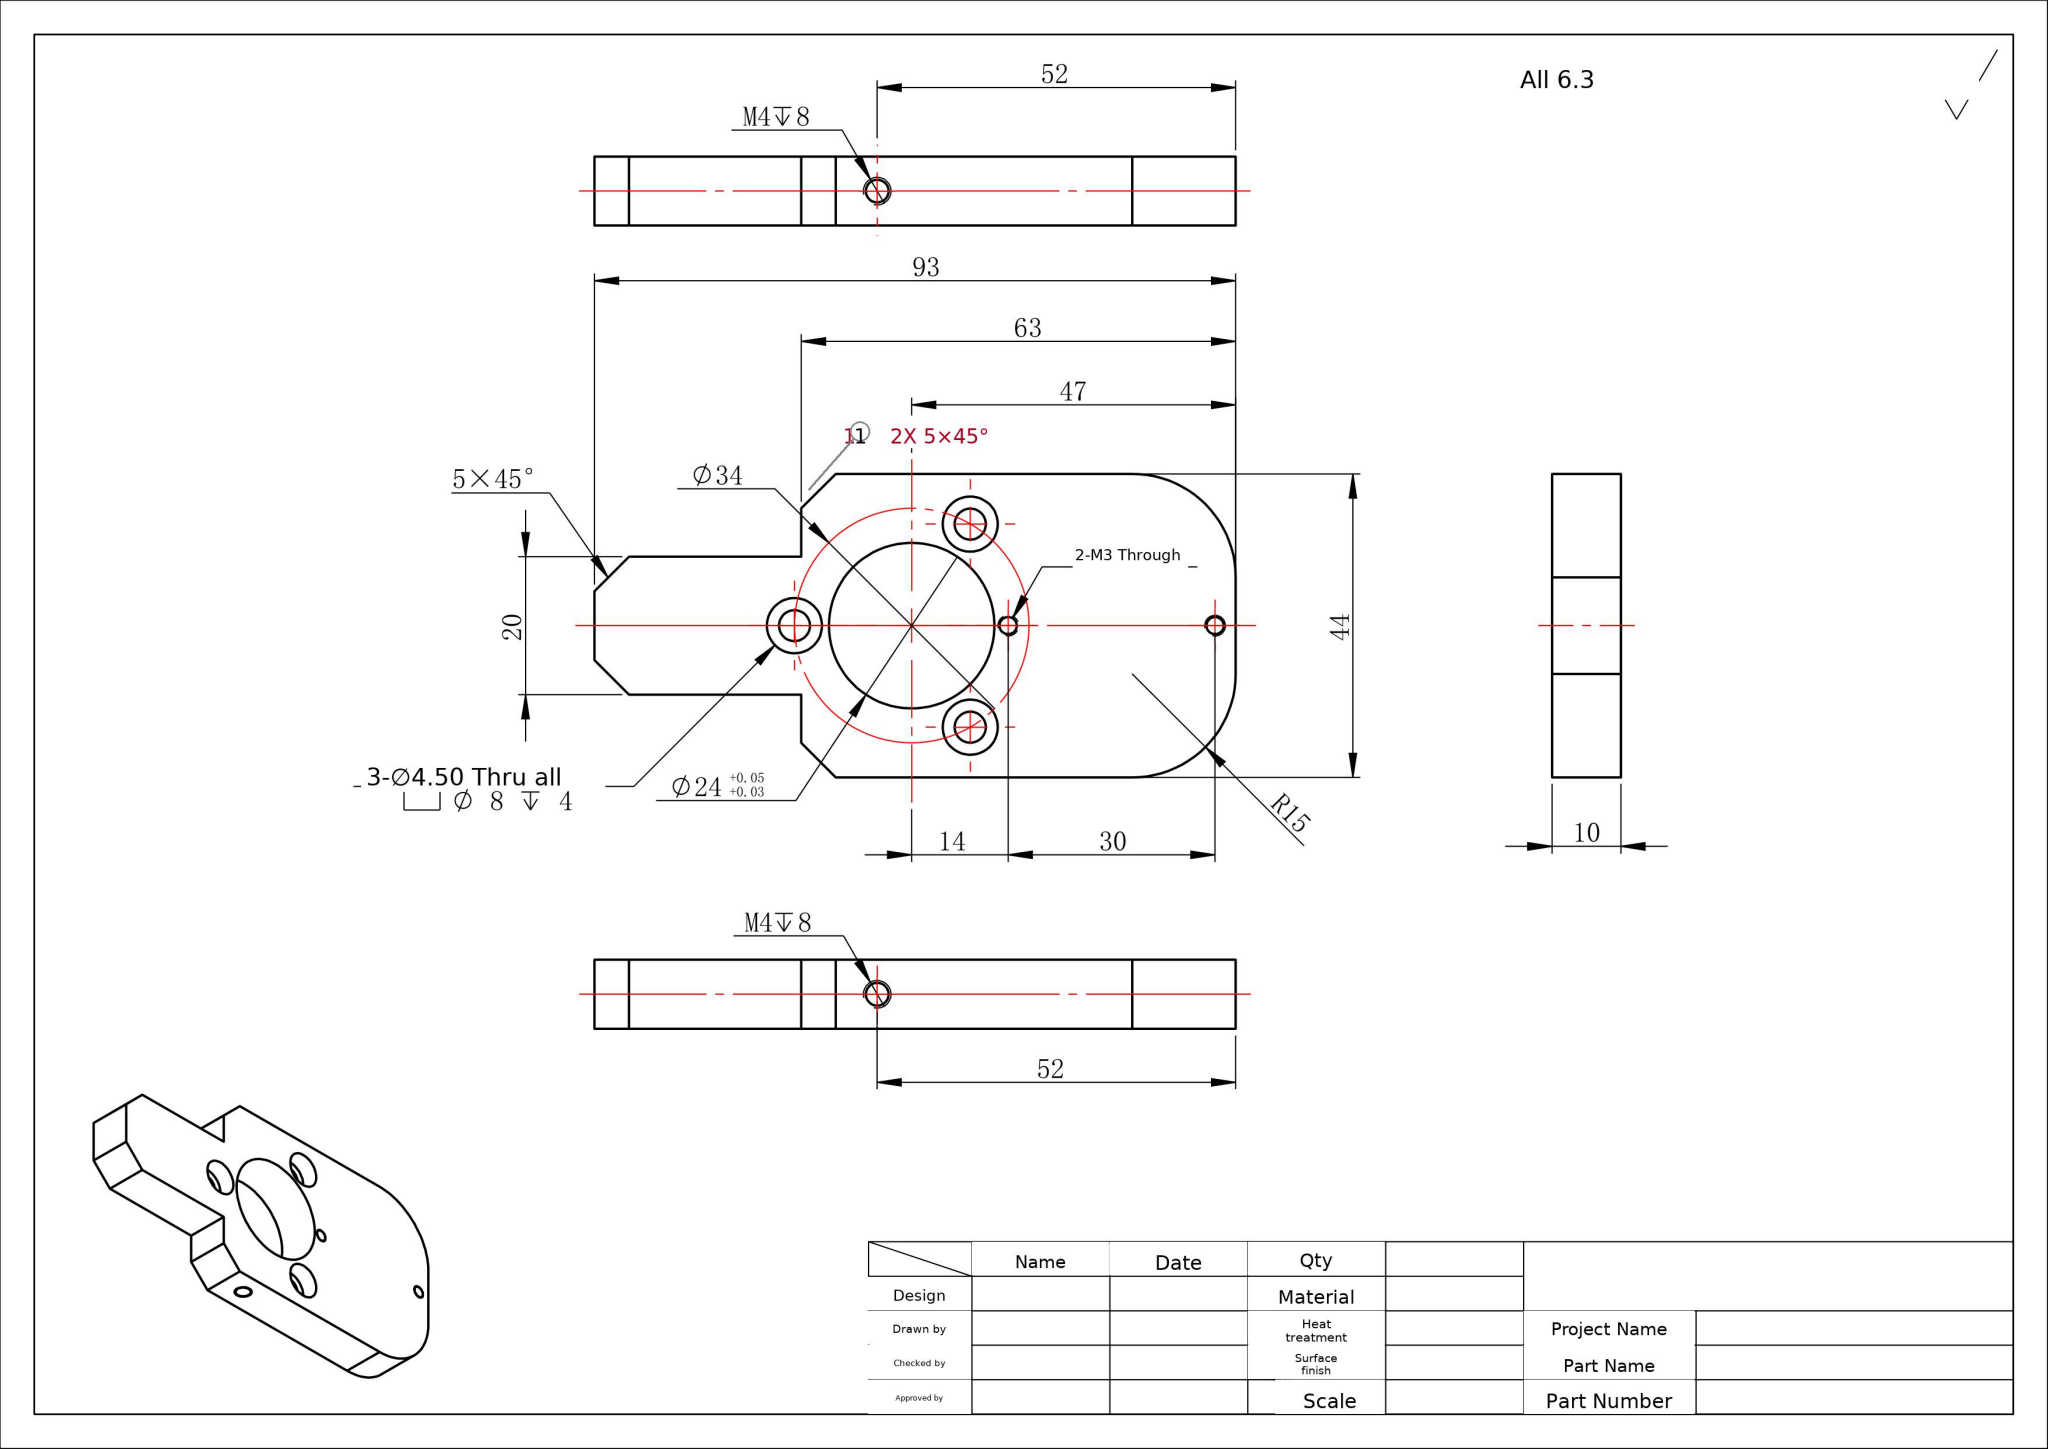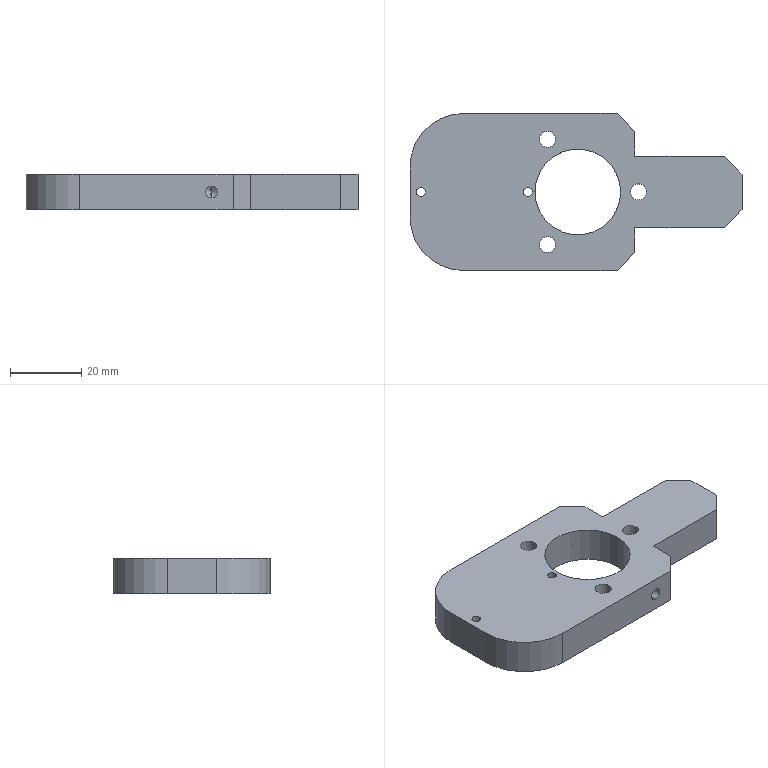Part | SolidWorks | mm | 1 solid | 45 faces | box 93 x 44 x 10 mm | volume 26566 mm3 | cylinder 24 | plane 17 | cone 4 | commonest cylinder face diameters 4.5 x6 8 x6 2.5 x4 3.3 x4 24 x2 30 x2
build123d program:
from build123d import *

# Parameters (mm, degrees)
SKETCH1_R                                       = 12
EXTRUDE1_DEPTH                                  = 10
SKETCH2_W                                       = 10
SKETCH2_H                                       = 20
EXTRUDE2_DEPTH                                  = 30
CHAMFER1_SIZE                                   = 5
CUT_EXTRUDE1_DEPTH                              = 54.716
M4_TAPPED_HOLE1_D                               = 3.3
M4_TAPPED_HOLE1_DEPTH                           = 10
M4_TAPPED_HOLE1_TIP                             = 0.9914
M4_TAPPED_HOLE2_D                               = 3.3
M4_TAPPED_HOLE2_DEPTH                           = 10
M4_TAPPED_HOLE2_TIP                             = 0.9914
M3_TAPPED_HOLE1_D                               = 2.5
M3_TAPPED_HOLE1_DEPTH                           = 11.5
M3_TAPPED_HOLE1_TIP                             = 0.7511
EXTRUDE3_DEPTH                                  = 10
SKETCH16_W                                      = 12.875
SKETCH16_H                                      = 46.518
CUT_EXTRUDE2_DEPTH                              = 53.938
M4_HEX_SOCKET_HEAD_CAP_SCREW_CBORE1_D           = 4.5
M4_HEX_SOCKET_HEAD_CAP_SCREW_CBORE1_CBORE_D     = 8
M4_HEX_SOCKET_HEAD_CAP_SCREW_CBORE1_CBORE_DEPTH = 4
FILLET1_R                                       = 15


with BuildPart() as part:
    # Sketch1 → Extrude1 (new body)
    with BuildSketch(Plane.XY):
        with BuildLine():
            Line((-42.635, -22), (16, -22))
            Line((16, -22), (16, 22))
            Line((16, 22), (-42.635, 22))
            ThreePointArc((-42.635, 22), (-47.973, 0), (-42.635, -22))
        make_face()
        Circle(SKETCH1_R, mode=Mode.SUBTRACT)
    extrude(amount=EXTRUDE1_DEPTH)

    # Sketch2 → Extrude2 (add)
    with BuildSketch(Plane(origin=(16, 0, 0), x_dir=(0, 0, -1), z_dir=(1, 0, 0))):
        with Locations((-5, 0)):
            Rectangle(SKETCH2_W, SKETCH2_H)
    extrude(amount=EXTRUDE2_DEPTH)

    # Chamfer1
    chamfer1_edges = [part.edges().sort_by_distance(p)[0] for p in [
        (46, -10, 5),
        (46, 10, 5),
        (16, -22, 5),
        (16, 22, 5),
    ]]
    chamfer(chamfer1_edges, length=CHAMFER1_SIZE)

    # Sketch8 → Cut-Extrude1 (cut, through all)
    with BuildSketch(Plane(origin=(0, 0, 0), x_dir=(-1, 0, 0), z_dir=(0, 0, -1))):
        with BuildLine():
            Line((37.98, 27.686), (49.876, 27.686))
            ThreePointArc((49.876, 27.686), (57.015, 1.842), (51.559, -24.409))
            Line((51.559, -24.409), (40.165, -24.409))
            ThreePointArc((40.165, -24.409), (46.959, 1.969), (37.98, 27.686))
        make_face()
    extrude(amount=-CUT_EXTRUDE1_DEPTH, mode=Mode.SUBTRACT)

    # M4 Tapped Hole1
    with Locations(Plane(origin=(5, -22, 5), x_dir=(0, 0, -1), z_dir=(0, -1, 0))):
        with Locations((0, 0)):
            Hole(M4_TAPPED_HOLE1_D / 2, depth=M4_TAPPED_HOLE1_DEPTH)
            with Locations((0, 0, -(M4_TAPPED_HOLE1_DEPTH + M4_TAPPED_HOLE1_TIP / 2))):  # 118° drill point
                Cone(0, M4_TAPPED_HOLE1_D / 2, M4_TAPPED_HOLE1_TIP, mode=Mode.SUBTRACT)

    # M4 Tapped Hole2
    with Locations(Plane(origin=(5, 22, 5), x_dir=(1, 0, 0), z_dir=(0, 1, 0))):
        with Locations((0, 0)):
            Hole(M4_TAPPED_HOLE2_D / 2, depth=M4_TAPPED_HOLE2_DEPTH)
            with Locations((0, 0, -(M4_TAPPED_HOLE2_DEPTH + M4_TAPPED_HOLE2_TIP / 2))):  # 118° drill point
                Cone(0, M4_TAPPED_HOLE2_D / 2, M4_TAPPED_HOLE2_TIP, mode=Mode.SUBTRACT)

    # M3 Tapped Hole1
    with Locations(Plane(origin=(-14, 0, 0), x_dir=(-1, 0, 0), z_dir=(0, 0, -1))):
        with Locations((0, 0), (30, 0)):
            Hole(M3_TAPPED_HOLE1_D / 2, depth=M3_TAPPED_HOLE1_DEPTH)
            with Locations((0, 0, -(M3_TAPPED_HOLE1_DEPTH + M3_TAPPED_HOLE1_TIP / 2))):  # 118° drill point
                Cone(0, M3_TAPPED_HOLE1_D / 2, M3_TAPPED_HOLE1_TIP, mode=Mode.SUBTRACT)

    # Sketch15 → Extrude3 (add)
    with BuildSketch(Plane(origin=(0, 0, 0), x_dir=(-1, 0, 0), z_dir=(0, 0, -1))):
        with BuildLine():
            Line((41.533, 22), (47.1, 22))
            Line((47.1, 22), (47.1, -22))
            Line((47.1, -22), (41.533, -22))
            ThreePointArc((41.533, -22), (47, 0), (41.533, 22))
        make_face()
    extrude(amount=-EXTRUDE3_DEPTH)

    # Sketch16 → Cut-Extrude2 (cut, through all)
    with BuildSketch(Plane(origin=(0, 0, 0), x_dir=(-1, 0, 0), z_dir=(0, 0, -1))):
        with Locations((53.437, 1.259)):
            Rectangle(SKETCH16_W, SKETCH16_H)
    extrude(amount=-CUT_EXTRUDE2_DEPTH, mode=Mode.SUBTRACT)

    # M4 Hex Socket Head Cap Screw CBORE1 (through all)
    with Locations(Plane(origin=(-8.5, 14.722, 0), x_dir=(-1, 0, 0), z_dir=(0, 0, -1))):
        with Locations((0, 0), (-25.5, -14.722), (0, -29.445)):
            CounterBoreHole(M4_HEX_SOCKET_HEAD_CAP_SCREW_CBORE1_D / 2, M4_HEX_SOCKET_HEAD_CAP_SCREW_CBORE1_CBORE_D / 2, M4_HEX_SOCKET_HEAD_CAP_SCREW_CBORE1_CBORE_DEPTH)

    # Fillet1
    fillet1_edges = [part.edges().sort_by_distance(p)[0] for p in [
        (-47, -22, 5),
        (-47, 22, 5),
    ]]
    fillet(fillet1_edges, radius=FILLET1_R)


solid = part.part